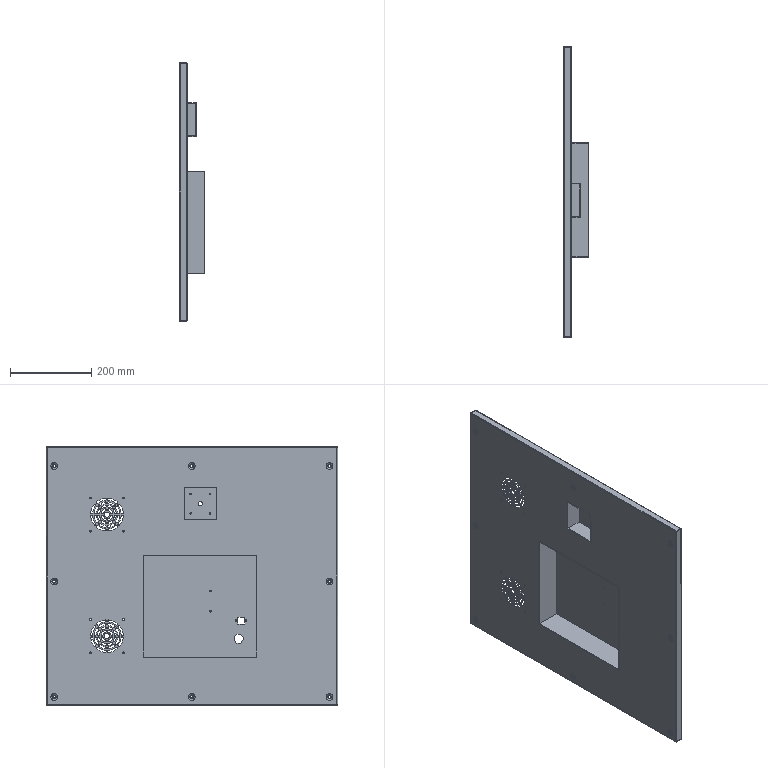Component | SolidWorks | 01-07RightGuardPlate-1 | 3 solids | 596 faces | volume 917045 mm3 | cylinder 388 | plane 104 | torus 64 | spline 40 | commonest cylinder face diameters 5 x168 4.5 x16 15 x16 12 x16 6.5 x16 71 x16 81 x16 54 x16 | material SPCC